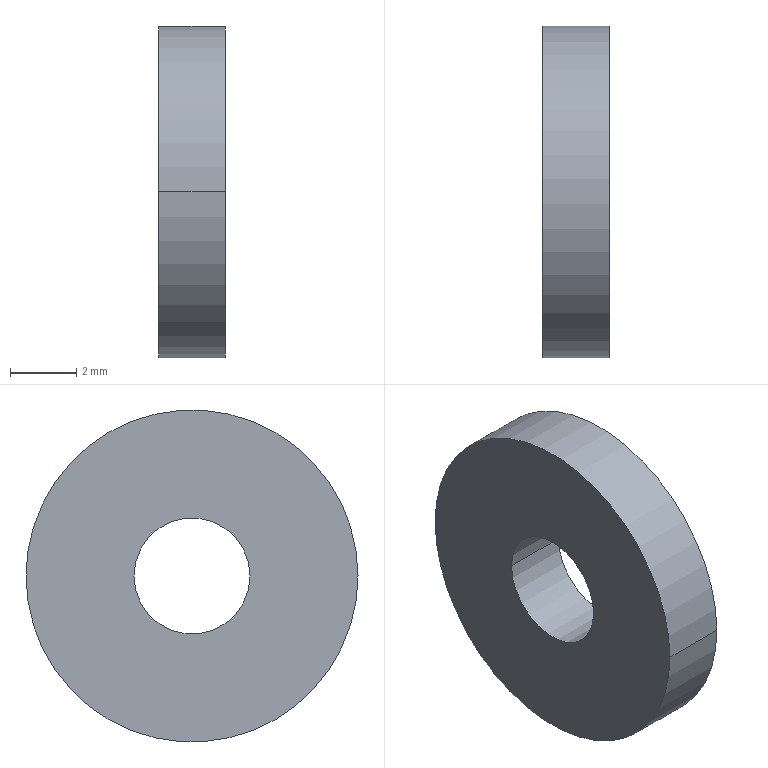Component | SolidWorks | ClampingArm2-1_A79-1 | 1 solid | 6 faces | box 2 x 10 x 10 mm | volume 138 mm3 | cylinder 4 | plane 2 | commonest cylinder face diameters 3.5 x2 10 x2 | material S45C
build123d program:
from build123d import *

# Parameters (mm, degrees)
SKETCH1_R           = 5
SKETCH1_R_2         = 1.75
BOSS_EXTRUDE1_DEPTH = 1


with BuildPart() as part:
    # Sketch1 → Boss-Extrude1 (new, symmetric)
    with BuildSketch(Plane(origin=(0, 0, 0), x_dir=(0, 0, -1), z_dir=(1, 0, 0))):
        Circle(SKETCH1_R)
        Circle(SKETCH1_R_2, mode=Mode.SUBTRACT)
    extrude(amount=BOSS_EXTRUDE1_DEPTH, both=True)


solid = part.part

# Placed as in the assembly
solid = solid.moved(Location((-1.551, 66.046, -22.5), (0, 0, 0)))
STEP:
#1=CARTESIAN_POINT('',(-0.02168,2.669,-0.8858));
#2=VERTEX_POINT('',#1);
#3=CARTESIAN_POINT('',(-0.02168,2.531,-0.8858));
#4=VERTEX_POINT('',#3);
#5=CARTESIAN_POINT('',(-0.02168,2.6,-0.8858));
#6=DIRECTION('',(1.,0.,-0.));
#7=DIRECTION('',(0.,-1.,0.0003333));
#8=AXIS2_PLACEMENT_3D('',#5,#6,#7);
#9=CIRCLE('',#8,0.0689);
#10=EDGE_CURVE('',#2,#4,#9,.T.);
#11=ORIENTED_EDGE('',*,*,#10,.T.);
#12=CARTESIAN_POINT('',(-0.1004,2.531,-0.8858));
#13=VERTEX_POINT('',#12);
#14=CARTESIAN_POINT('',(-0.02168,2.531,-0.8858));
#15=DIRECTION('',(-1.,-0.,0.));
#16=VECTOR('',#15,39.37);
#17=LINE('',#14,#16);
#18=EDGE_CURVE('',#4,#13,#17,.T.);
#19=ORIENTED_EDGE('',*,*,#18,.T.);
#20=CARTESIAN_POINT('',(-0.1004,2.669,-0.8858));
#21=VERTEX_POINT('',#20);
#22=CARTESIAN_POINT('',(-0.1004,2.6,-0.8858));
#23=DIRECTION('',(1.,0.,-0.));
#24=DIRECTION('',(0.,-1.,0.0003333));
#25=AXIS2_PLACEMENT_3D('',#22,#23,#24);
#26=CIRCLE('',#25,0.0689);
#27=EDGE_CURVE('',#21,#13,#26,.T.);
#28=ORIENTED_EDGE('',*,*,#27,.F.);
#29=CARTESIAN_POINT('',(-0.02168,2.669,-0.8858));
#30=DIRECTION('',(-1.,-0.,0.));
#31=VECTOR('',#30,39.37);
#32=LINE('',#29,#31);
#33=EDGE_CURVE('',#2,#21,#32,.T.);
#34=ORIENTED_EDGE('',*,*,#33,.F.);
#35=EDGE_LOOP('',(#11,#19,#28,#34));
#36=FACE_OUTER_BOUND('',#35,.T.);
#37=CARTESIAN_POINT('',(-0.02168,2.6,-0.8858));
#38=DIRECTION('',(-1.,-0.,0.));
#39=DIRECTION('',(0.,1.,-0.0003333));
#40=AXIS2_PLACEMENT_3D('',#37,#38,#39);
#41=CYLINDRICAL_SURFACE('',#40,0.0689);
#42=ADVANCED_FACE('',(#36),#41,.F.);
#43=CARTESIAN_POINT('',(-0.02168,2.403,-0.8858));
#44=VERTEX_POINT('',#43);
#45=CARTESIAN_POINT('',(-0.02168,2.797,-0.8859));
#46=VERTEX_POINT('',#45);
#47=CARTESIAN_POINT('',(-0.02168,2.6,-0.8858));
#48=DIRECTION('',(1.,0.,-0.));
#49=DIRECTION('',(0.,-1.,0.0003333));
#50=AXIS2_PLACEMENT_3D('',#47,#48,#49);
#51=CIRCLE('',#50,0.1969);
#52=EDGE_CURVE('',#44,#46,#51,.T.);
#53=ORIENTED_EDGE('',*,*,#52,.F.);
#54=CARTESIAN_POINT('',(-0.1004,2.403,-0.8858));
#55=VERTEX_POINT('',#54);
#56=CARTESIAN_POINT('',(-0.02168,2.403,-0.8858));
#57=DIRECTION('',(-1.,-0.,0.));
#58=VECTOR('',#57,39.37);
#59=LINE('',#56,#58);
#60=EDGE_CURVE('',#44,#55,#59,.T.);
#61=ORIENTED_EDGE('',*,*,#60,.T.);
#62=CARTESIAN_POINT('',(-0.1004,2.797,-0.8859));
#63=VERTEX_POINT('',#62);
#64=CARTESIAN_POINT('',(-0.1004,2.6,-0.8858));
#65=DIRECTION('',(1.,0.,-0.));
#66=DIRECTION('',(0.,-1.,0.0003333));
#67=AXIS2_PLACEMENT_3D('',#64,#65,#66);
#68=CIRCLE('',#67,0.1969);
#69=EDGE_CURVE('',#55,#63,#68,.T.);
#70=ORIENTED_EDGE('',*,*,#69,.T.);
#71=CARTESIAN_POINT('',(-0.02168,2.797,-0.8859));
#72=DIRECTION('',(-1.,-0.,0.));
#73=VECTOR('',#72,39.37);
#74=LINE('',#71,#73);
#75=EDGE_CURVE('',#46,#63,#74,.T.);
#76=ORIENTED_EDGE('',*,*,#75,.F.);
#77=EDGE_LOOP('',(#53,#61,#70,#76));
#78=FACE_OUTER_BOUND('',#77,.T.);
#79=CARTESIAN_POINT('',(-0.02168,2.6,-0.8858));
#80=DIRECTION('',(-1.,-0.,0.));
#81=DIRECTION('',(0.,1.,-0.0003333));
#82=AXIS2_PLACEMENT_3D('',#79,#80,#81);
#83=CYLINDRICAL_SURFACE('',#82,0.1969);
#84=ADVANCED_FACE('',(#78),#83,.T.);
#85=CARTESIAN_POINT('',(-0.02168,2.6,-0.8858));
#86=DIRECTION('',(1.,0.,-0.));
#87=DIRECTION('',(0.,-1.,0.0003333));
#88=AXIS2_PLACEMENT_3D('',#85,#86,#87);
#89=CIRCLE('',#88,0.1969);
#90=EDGE_CURVE('',#46,#44,#89,.T.);
#91=ORIENTED_EDGE('',*,*,#90,.T.);
#92=ORIENTED_EDGE('',*,*,#52,.T.);
#93=EDGE_LOOP('',(#91,#92));
#94=FACE_OUTER_BOUND('',#93,.T.);
#95=ORIENTED_EDGE('',*,*,#10,.F.);
#96=CARTESIAN_POINT('',(-0.02168,2.6,-0.8858));
#97=DIRECTION('',(1.,0.,-0.));
#98=DIRECTION('',(0.,-1.,0.0003333));
#99=AXIS2_PLACEMENT_3D('',#96,#97,#98);
#100=CIRCLE('',#99,0.0689);
#101=EDGE_CURVE('',#4,#2,#100,.T.);
#102=ORIENTED_EDGE('',*,*,#101,.F.);
#103=EDGE_LOOP('',(#95,#102));
#104=FACE_BOUND('',#103,.T.);
#105=CARTESIAN_POINT('',(-0.02168,2.6,-0.8858));
#106=DIRECTION('',(1.,0.,-0.));
#107=DIRECTION('',(0.,-1.,0.0003333));
#108=AXIS2_PLACEMENT_3D('',#105,#106,#107);
#109=PLANE('',#108);
#110=ADVANCED_FACE('',(#94,#104),#109,.T.);
#111=CARTESIAN_POINT('',(-0.1004,2.6,-0.8858));
#112=DIRECTION('',(1.,0.,-0.));
#113=DIRECTION('',(0.,-1.,0.0003333));
#114=AXIS2_PLACEMENT_3D('',#111,#112,#113);
#115=CIRCLE('',#114,0.1969);
#116=EDGE_CURVE('',#63,#55,#115,.T.);
#117=ORIENTED_EDGE('',*,*,#116,.F.);
#118=ORIENTED_EDGE('',*,*,#69,.F.);
#119=EDGE_LOOP('',(#117,#118));
#120=FACE_OUTER_BOUND('',#119,.T.);
#121=ORIENTED_EDGE('',*,*,#27,.T.);
#122=CARTESIAN_POINT('',(-0.1004,2.6,-0.8858));
#123=DIRECTION('',(1.,0.,-0.));
#124=DIRECTION('',(0.,-1.,0.0003333));
#125=AXIS2_PLACEMENT_3D('',#122,#123,#124);
#126=CIRCLE('',#125,0.0689);
#127=EDGE_CURVE('',#13,#21,#126,.T.);
#128=ORIENTED_EDGE('',*,*,#127,.T.);
#129=EDGE_LOOP('',(#121,#128));
#130=FACE_BOUND('',#129,.T.);
#131=CARTESIAN_POINT('',(-0.1004,2.6,-0.8858));
#132=DIRECTION('',(1.,0.,-0.));
#133=DIRECTION('',(0.,-1.,0.0003333));
#134=AXIS2_PLACEMENT_3D('',#131,#132,#133);
#135=PLANE('',#134);
#136=ADVANCED_FACE('',(#120,#130),#135,.F.);
#137=ORIENTED_EDGE('',*,*,#60,.F.);
#138=ORIENTED_EDGE('',*,*,#90,.F.);
#139=ORIENTED_EDGE('',*,*,#75,.T.);
#140=ORIENTED_EDGE('',*,*,#116,.T.);
#141=EDGE_LOOP('',(#137,#138,#139,#140));
#142=FACE_OUTER_BOUND('',#141,.T.);
#143=CARTESIAN_POINT('',(-0.02168,2.6,-0.8858));
#144=DIRECTION('',(-1.,-0.,0.));
#145=DIRECTION('',(0.,1.,-0.0003333));
#146=AXIS2_PLACEMENT_3D('',#143,#144,#145);
#147=CYLINDRICAL_SURFACE('',#146,0.1969);
#148=ADVANCED_FACE('',(#142),#147,.T.);
#149=ORIENTED_EDGE('',*,*,#18,.F.);
#150=ORIENTED_EDGE('',*,*,#101,.T.);
#151=ORIENTED_EDGE('',*,*,#33,.T.);
#152=ORIENTED_EDGE('',*,*,#127,.F.);
#153=EDGE_LOOP('',(#149,#150,#151,#152));
#154=FACE_OUTER_BOUND('',#153,.T.);
#155=CARTESIAN_POINT('',(-0.02168,2.6,-0.8858));
#156=DIRECTION('',(-1.,-0.,0.));
#157=DIRECTION('',(0.,1.,-0.0003333));
#158=AXIS2_PLACEMENT_3D('',#155,#156,#157);
#159=CYLINDRICAL_SURFACE('',#158,0.0689);
#160=ADVANCED_FACE('',(#154),#159,.F.);
#161=CLOSED_SHELL('',(#42,#84,#110,#136,#148,#160));
#162=MANIFOLD_SOLID_BREP('',#161);
#163=CARTESIAN_POINT('',(0.,0.,0.));
#164=DIRECTION('',(0.,0.,1.));
#165=DIRECTION('',(1.,0.,0.));
#166=AXIS2_PLACEMENT_3D('',#163,#164,#165);
#167=(LENGTH_UNIT()NAMED_UNIT(*)SI_UNIT($,.METRE.));
#168=LENGTH_MEASURE_WITH_UNIT(LENGTH_MEASURE(0.0254),#167);
#169=DIMENSIONAL_EXPONENTS(1.,0.,0.,0.,0.,0.,0.);
#170=(CONVERSION_BASED_UNIT('',#168)LENGTH_UNIT()NAMED_UNIT(#169));
#171=UNCERTAINTY_MEASURE_WITH_UNIT(LENGTH_MEASURE(0.00001),#170,'','');
#172=(NAMED_UNIT(*)PLANE_ANGLE_UNIT()SI_UNIT($,.RADIAN.));
#173=(NAMED_UNIT(*)SI_UNIT($,.STERADIAN.)SOLID_ANGLE_UNIT());
#174=(GEOMETRIC_REPRESENTATION_CONTEXT(3)GLOBAL_UNCERTAINTY_ASSIGNED_CONTEXT((#171))GLOBAL_UNIT_ASSIGNED_CONTEXT((#170,#172,#173))REPRESENTATION_CONTEXT('',''));
#175=ADVANCED_BREP_SHAPE_REPRESENTATION('',(#162,#166),#174);
#176=COLOUR_RGB('',0.7922,0.8196,0.9333);
#177=FILL_AREA_STYLE_COLOUR('',#176);
#178=FILL_AREA_STYLE('',(#177));
#179=SURFACE_STYLE_FILL_AREA(#178);
#180=SURFACE_SIDE_STYLE('',(#179));
#181=SURFACE_STYLE_USAGE(.BOTH.,#180);
#182=PRESENTATION_STYLE_ASSIGNMENT((#181));
#183=STYLED_ITEM('',(#182),#162);
#184=PRESENTATION_LAYER_ASSIGNMENT('','',(#183));
#185=(LENGTH_UNIT()NAMED_UNIT(*)SI_UNIT($,.METRE.));
#186=LENGTH_MEASURE_WITH_UNIT(LENGTH_MEASURE(0.0254),#185);
#187=DIMENSIONAL_EXPONENTS(1.,0.,0.,0.,0.,0.,0.);
#188=(CONVERSION_BASED_UNIT('',#186)LENGTH_UNIT()NAMED_UNIT(#187));
#189=UNCERTAINTY_MEASURE_WITH_UNIT(LENGTH_MEASURE(0.00001),#188,'','');
#190=(NAMED_UNIT(*)PLANE_ANGLE_UNIT()SI_UNIT($,.RADIAN.));
#191=(NAMED_UNIT(*)SI_UNIT($,.STERADIAN.)SOLID_ANGLE_UNIT());
#192=(GEOMETRIC_REPRESENTATION_CONTEXT(3)GLOBAL_UNCERTAINTY_ASSIGNED_CONTEXT((#189))GLOBAL_UNIT_ASSIGNED_CONTEXT((#188,#190,#191))REPRESENTATION_CONTEXT('',''));
#193=MECHANICAL_DESIGN_GEOMETRIC_PRESENTATION_REPRESENTATION('',(#183),#192);